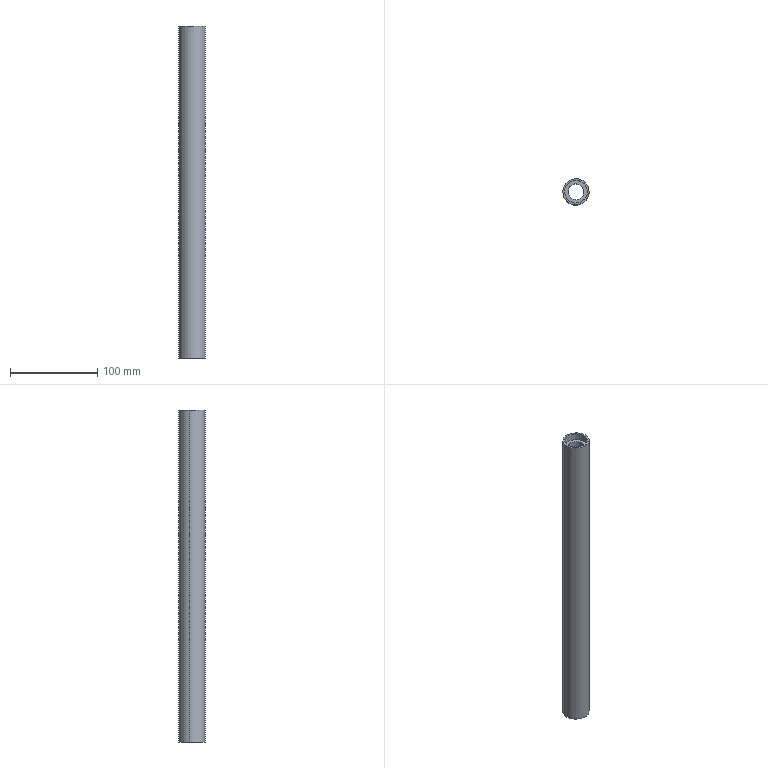Component | SolidWorks | Roller1-2-1_Roller1-1 | 1 solid | 12 faces | box 30 x 30 x 380 mm | volume 167485 mm3 | cylinder 8 | plane 4 | commonest cylinder face diameters 26 x4 18 x2 30 x2
build123d program:
from build123d import *


with BuildPart() as part:
    # Sketch1 → Revolve1 (revolve)
    with BuildSketch(Plane(origin=(0, 0, 0), x_dir=(-1, 0, 0), z_dir=(0, 0, -1)), mode=Mode.PRIVATE) as revolve1_sk:
        Polygon((-182, 13), (-182, 9), (182, 9), (182, 13), (190, 13), (190, 15), (-190, 15), (-190, 13), align=None)
    revolve(revolve1_sk.sketch.rotate(Axis((190, 0, 0), (-1, 0, 0)), 270), axis=Axis((190, 0, 0), (-1, 0, 0)))


solid = part.part

# Placed as in the assembly
solid = solid.moved(Location((-365, 591, 0), (0, 90, 0)))
STEP:
#1=CARTESIAN_POINT('',(-14.024,23.192,-7.165));
#2=VERTEX_POINT('',#1);
#3=CARTESIAN_POINT('',(-14.716,23.344,-7.165));
#4=VERTEX_POINT('',#3);
#5=CARTESIAN_POINT('',(-14.37,23.268,-7.165));
#6=DIRECTION('',(-0.,0.,1.));
#7=DIRECTION('',(-0.9768,0.2142,0.));
#8=AXIS2_PLACEMENT_3D('',#5,#6,#7);
#9=CIRCLE('',#8,0.3543);
#10=EDGE_CURVE('',#2,#4,#9,.T.);
#11=ORIENTED_EDGE('',*,*,#10,.F.);
#12=CARTESIAN_POINT('',(-14.024,23.192,7.165));
#13=VERTEX_POINT('',#12);
#14=CARTESIAN_POINT('',(-14.024,23.192,-7.48));
#15=DIRECTION('',(-0.,0.,1.));
#16=VECTOR('',#15,39.37);
#17=LINE('',#14,#16);
#18=EDGE_CURVE('',#2,#13,#17,.T.);
#19=ORIENTED_EDGE('',*,*,#18,.T.);
#20=CARTESIAN_POINT('',(-14.716,23.344,7.165));
#21=VERTEX_POINT('',#20);
#22=CARTESIAN_POINT('',(-14.37,23.268,7.165));
#23=DIRECTION('',(-0.,0.,1.));
#24=DIRECTION('',(-0.9768,0.2142,0.));
#25=AXIS2_PLACEMENT_3D('',#22,#23,#24);
#26=CIRCLE('',#25,0.3543);
#27=EDGE_CURVE('',#13,#21,#26,.T.);
#28=ORIENTED_EDGE('',*,*,#27,.T.);
#29=CARTESIAN_POINT('',(-14.716,23.344,-7.48));
#30=DIRECTION('',(-0.,0.,1.));
#31=VECTOR('',#30,39.37);
#32=LINE('',#29,#31);
#33=EDGE_CURVE('',#4,#21,#32,.T.);
#34=ORIENTED_EDGE('',*,*,#33,.F.);
#35=EDGE_LOOP('',(#11,#19,#28,#34));
#36=FACE_OUTER_BOUND('',#35,.T.);
#37=CARTESIAN_POINT('',(-14.37,23.268,-7.48));
#38=DIRECTION('',(-0.,0.,1.));
#39=DIRECTION('',(-0.9768,0.2142,0.));
#40=AXIS2_PLACEMENT_3D('',#37,#38,#39);
#41=CYLINDRICAL_SURFACE('',#40,0.3543);
#42=ADVANCED_FACE('',(#36),#41,.F.);
#43=CARTESIAN_POINT('',(-13.87,23.158,7.165));
#44=VERTEX_POINT('',#43);
#45=CARTESIAN_POINT('',(-14.87,23.377,7.165));
#46=VERTEX_POINT('',#45);
#47=CARTESIAN_POINT('',(-14.37,23.268,7.165));
#48=DIRECTION('',(-0.,0.,1.));
#49=DIRECTION('',(-0.9768,0.2142,0.));
#50=AXIS2_PLACEMENT_3D('',#47,#48,#49);
#51=CIRCLE('',#50,0.5118);
#52=EDGE_CURVE('',#44,#46,#51,.T.);
#53=ORIENTED_EDGE('',*,*,#52,.F.);
#54=CARTESIAN_POINT('',(-13.87,23.158,7.48));
#55=VERTEX_POINT('',#54);
#56=CARTESIAN_POINT('',(-13.87,23.158,-7.48));
#57=DIRECTION('',(-0.,0.,1.));
#58=VECTOR('',#57,39.37);
#59=LINE('',#56,#58);
#60=EDGE_CURVE('',#44,#55,#59,.T.);
#61=ORIENTED_EDGE('',*,*,#60,.T.);
#62=CARTESIAN_POINT('',(-14.87,23.377,7.48));
#63=VERTEX_POINT('',#62);
#64=CARTESIAN_POINT('',(-14.37,23.268,7.48));
#65=DIRECTION('',(-0.,0.,1.));
#66=DIRECTION('',(-0.9768,0.2142,0.));
#67=AXIS2_PLACEMENT_3D('',#64,#65,#66);
#68=CIRCLE('',#67,0.5118);
#69=EDGE_CURVE('',#55,#63,#68,.T.);
#70=ORIENTED_EDGE('',*,*,#69,.T.);
#71=CARTESIAN_POINT('',(-14.87,23.377,-7.48));
#72=DIRECTION('',(-0.,0.,1.));
#73=VECTOR('',#72,39.37);
#74=LINE('',#71,#73);
#75=EDGE_CURVE('',#46,#63,#74,.T.);
#76=ORIENTED_EDGE('',*,*,#75,.F.);
#77=EDGE_LOOP('',(#53,#61,#70,#76));
#78=FACE_OUTER_BOUND('',#77,.T.);
#79=CARTESIAN_POINT('',(-14.37,23.268,-7.48));
#80=DIRECTION('',(-0.,0.,1.));
#81=DIRECTION('',(-0.9768,0.2142,0.));
#82=AXIS2_PLACEMENT_3D('',#79,#80,#81);
#83=CYLINDRICAL_SURFACE('',#82,0.5118);
#84=ADVANCED_FACE('',(#78),#83,.F.);
#85=CARTESIAN_POINT('',(-14.947,23.394,-7.48));
#86=VERTEX_POINT('',#85);
#87=CARTESIAN_POINT('',(-13.793,23.141,-7.48));
#88=VERTEX_POINT('',#87);
#89=CARTESIAN_POINT('',(-14.37,23.268,-7.48));
#90=DIRECTION('',(-0.,0.,1.));
#91=DIRECTION('',(-0.9768,0.2142,0.));
#92=AXIS2_PLACEMENT_3D('',#89,#90,#91);
#93=CIRCLE('',#92,0.5906);
#94=EDGE_CURVE('',#86,#88,#93,.T.);
#95=ORIENTED_EDGE('',*,*,#94,.T.);
#96=CARTESIAN_POINT('',(-13.793,23.141,7.48));
#97=VERTEX_POINT('',#96);
#98=CARTESIAN_POINT('',(-13.793,23.141,-7.48));
#99=DIRECTION('',(-0.,0.,1.));
#100=VECTOR('',#99,39.37);
#101=LINE('',#98,#100);
#102=EDGE_CURVE('',#88,#97,#101,.T.);
#103=ORIENTED_EDGE('',*,*,#102,.T.);
#104=CARTESIAN_POINT('',(-14.947,23.394,7.48));
#105=VERTEX_POINT('',#104);
#106=CARTESIAN_POINT('',(-14.37,23.268,7.48));
#107=DIRECTION('',(-0.,0.,1.));
#108=DIRECTION('',(-0.9768,0.2142,0.));
#109=AXIS2_PLACEMENT_3D('',#106,#107,#108);
#110=CIRCLE('',#109,0.5906);
#111=EDGE_CURVE('',#105,#97,#110,.T.);
#112=ORIENTED_EDGE('',*,*,#111,.F.);
#113=CARTESIAN_POINT('',(-14.947,23.394,-7.48));
#114=DIRECTION('',(-0.,0.,1.));
#115=VECTOR('',#114,39.37);
#116=LINE('',#113,#115);
#117=EDGE_CURVE('',#86,#105,#116,.T.);
#118=ORIENTED_EDGE('',*,*,#117,.F.);
#119=EDGE_LOOP('',(#95,#103,#112,#118));
#120=FACE_OUTER_BOUND('',#119,.T.);
#121=CARTESIAN_POINT('',(-14.37,23.268,-7.48));
#122=DIRECTION('',(-0.,0.,1.));
#123=DIRECTION('',(-0.9768,0.2142,0.));
#124=AXIS2_PLACEMENT_3D('',#121,#122,#123);
#125=CYLINDRICAL_SURFACE('',#124,0.5906);
#126=ADVANCED_FACE('',(#120),#125,.T.);
#127=CARTESIAN_POINT('',(-13.87,23.158,-7.48));
#128=VERTEX_POINT('',#127);
#129=CARTESIAN_POINT('',(-14.87,23.377,-7.48));
#130=VERTEX_POINT('',#129);
#131=CARTESIAN_POINT('',(-14.37,23.268,-7.48));
#132=DIRECTION('',(-0.,0.,1.));
#133=DIRECTION('',(-0.9768,0.2142,0.));
#134=AXIS2_PLACEMENT_3D('',#131,#132,#133);
#135=CIRCLE('',#134,0.5118);
#136=EDGE_CURVE('',#128,#130,#135,.T.);
#137=ORIENTED_EDGE('',*,*,#136,.F.);
#138=CARTESIAN_POINT('',(-13.87,23.158,-7.165));
#139=VERTEX_POINT('',#138);
#140=CARTESIAN_POINT('',(-13.87,23.158,-7.48));
#141=DIRECTION('',(-0.,0.,1.));
#142=VECTOR('',#141,39.37);
#143=LINE('',#140,#142);
#144=EDGE_CURVE('',#128,#139,#143,.T.);
#145=ORIENTED_EDGE('',*,*,#144,.T.);
#146=CARTESIAN_POINT('',(-14.87,23.377,-7.165));
#147=VERTEX_POINT('',#146);
#148=CARTESIAN_POINT('',(-14.37,23.268,-7.165));
#149=DIRECTION('',(-0.,0.,1.));
#150=DIRECTION('',(-0.9768,0.2142,0.));
#151=AXIS2_PLACEMENT_3D('',#148,#149,#150);
#152=CIRCLE('',#151,0.5118);
#153=EDGE_CURVE('',#139,#147,#152,.T.);
#154=ORIENTED_EDGE('',*,*,#153,.T.);
#155=CARTESIAN_POINT('',(-14.87,23.377,-7.48));
#156=DIRECTION('',(-0.,0.,1.));
#157=VECTOR('',#156,39.37);
#158=LINE('',#155,#157);
#159=EDGE_CURVE('',#130,#147,#158,.T.);
#160=ORIENTED_EDGE('',*,*,#159,.F.);
#161=EDGE_LOOP('',(#137,#145,#154,#160));
#162=FACE_OUTER_BOUND('',#161,.T.);
#163=CARTESIAN_POINT('',(-14.37,23.268,-7.48));
#164=DIRECTION('',(-0.,0.,1.));
#165=DIRECTION('',(-0.9768,0.2142,0.));
#166=AXIS2_PLACEMENT_3D('',#163,#164,#165);
#167=CYLINDRICAL_SURFACE('',#166,0.5118);
#168=ADVANCED_FACE('',(#162),#167,.F.);
#169=ORIENTED_EDGE('',*,*,#144,.F.);
#170=CARTESIAN_POINT('',(-14.37,23.268,-7.48));
#171=DIRECTION('',(-0.,0.,1.));
#172=DIRECTION('',(-0.9768,0.2142,0.));
#173=AXIS2_PLACEMENT_3D('',#170,#171,#172);
#174=CIRCLE('',#173,0.5118);
#175=EDGE_CURVE('',#130,#128,#174,.T.);
#176=ORIENTED_EDGE('',*,*,#175,.F.);
#177=ORIENTED_EDGE('',*,*,#159,.T.);
#178=CARTESIAN_POINT('',(-14.37,23.268,-7.165));
#179=DIRECTION('',(-0.,0.,1.));
#180=DIRECTION('',(-0.9768,0.2142,0.));
#181=AXIS2_PLACEMENT_3D('',#178,#179,#180);
#182=CIRCLE('',#181,0.5118);
#183=EDGE_CURVE('',#147,#139,#182,.T.);
#184=ORIENTED_EDGE('',*,*,#183,.T.);
#185=EDGE_LOOP('',(#169,#176,#177,#184));
#186=FACE_OUTER_BOUND('',#185,.T.);
#187=CARTESIAN_POINT('',(-14.37,23.268,-7.48));
#188=DIRECTION('',(-0.,0.,1.));
#189=DIRECTION('',(-0.9768,0.2142,0.));
#190=AXIS2_PLACEMENT_3D('',#187,#188,#189);
#191=CYLINDRICAL_SURFACE('',#190,0.5118);
#192=ADVANCED_FACE('',(#186),#191,.F.);
#193=ORIENTED_EDGE('',*,*,#175,.T.);
#194=ORIENTED_EDGE('',*,*,#136,.T.);
#195=EDGE_LOOP('',(#193,#194));
#196=FACE_BOUND('',#195,.T.);
#197=ORIENTED_EDGE('',*,*,#94,.F.);
#198=CARTESIAN_POINT('',(-14.37,23.268,-7.48));
#199=DIRECTION('',(-0.,0.,1.));
#200=DIRECTION('',(-0.9768,0.2142,0.));
#201=AXIS2_PLACEMENT_3D('',#198,#199,#200);
#202=CIRCLE('',#201,0.5906);
#203=EDGE_CURVE('',#88,#86,#202,.T.);
#204=ORIENTED_EDGE('',*,*,#203,.F.);
#205=EDGE_LOOP('',(#197,#204));
#206=FACE_OUTER_BOUND('',#205,.T.);
#207=CARTESIAN_POINT('',(-14.497,22.691,-7.48));
#208=DIRECTION('',(0.,-0.,-1.));
#209=DIRECTION('',(0.9768,-0.2142,0.));
#210=AXIS2_PLACEMENT_3D('',#207,#208,#209);
#211=PLANE('',#210);
#212=ADVANCED_FACE('',(#196,#206),#211,.T.);
#213=ORIENTED_EDGE('',*,*,#102,.F.);
#214=ORIENTED_EDGE('',*,*,#203,.T.);
#215=ORIENTED_EDGE('',*,*,#117,.T.);
#216=CARTESIAN_POINT('',(-14.37,23.268,7.48));
#217=DIRECTION('',(-0.,0.,1.));
#218=DIRECTION('',(-0.9768,0.2142,0.));
#219=AXIS2_PLACEMENT_3D('',#216,#217,#218);
#220=CIRCLE('',#219,0.5906);
#221=EDGE_CURVE('',#97,#105,#220,.T.);
#222=ORIENTED_EDGE('',*,*,#221,.F.);
#223=EDGE_LOOP('',(#213,#214,#215,#222));
#224=FACE_OUTER_BOUND('',#223,.T.);
#225=CARTESIAN_POINT('',(-14.37,23.268,-7.48));
#226=DIRECTION('',(-0.,0.,1.));
#227=DIRECTION('',(-0.9768,0.2142,0.));
#228=AXIS2_PLACEMENT_3D('',#225,#226,#227);
#229=CYLINDRICAL_SURFACE('',#228,0.5906);
#230=ADVANCED_FACE('',(#224),#229,.T.);
#231=ORIENTED_EDGE('',*,*,#111,.T.);
#232=ORIENTED_EDGE('',*,*,#221,.T.);
#233=EDGE_LOOP('',(#231,#232));
#234=FACE_OUTER_BOUND('',#233,.T.);
#235=CARTESIAN_POINT('',(-14.37,23.268,7.48));
#236=DIRECTION('',(-0.,0.,1.));
#237=DIRECTION('',(-0.9768,0.2142,0.));
#238=AXIS2_PLACEMENT_3D('',#235,#236,#237);
#239=CIRCLE('',#238,0.5118);
#240=EDGE_CURVE('',#63,#55,#239,.T.);
#241=ORIENTED_EDGE('',*,*,#240,.F.);
#242=ORIENTED_EDGE('',*,*,#69,.F.);
#243=EDGE_LOOP('',(#241,#242));
#244=FACE_BOUND('',#243,.T.);
#245=CARTESIAN_POINT('',(-14.48,22.768,7.48));
#246=DIRECTION('',(-0.,0.,1.));
#247=DIRECTION('',(-0.9768,0.2142,-0.));
#248=AXIS2_PLACEMENT_3D('',#245,#246,#247);
#249=PLANE('',#248);
#250=ADVANCED_FACE('',(#234,#244),#249,.T.);
#251=ORIENTED_EDGE('',*,*,#60,.F.);
#252=CARTESIAN_POINT('',(-14.37,23.268,7.165));
#253=DIRECTION('',(-0.,0.,1.));
#254=DIRECTION('',(-0.9768,0.2142,0.));
#255=AXIS2_PLACEMENT_3D('',#252,#253,#254);
#256=CIRCLE('',#255,0.5118);
#257=EDGE_CURVE('',#46,#44,#256,.T.);
#258=ORIENTED_EDGE('',*,*,#257,.F.);
#259=ORIENTED_EDGE('',*,*,#75,.T.);
#260=ORIENTED_EDGE('',*,*,#240,.T.);
#261=EDGE_LOOP('',(#251,#258,#259,#260));
#262=FACE_OUTER_BOUND('',#261,.T.);
#263=CARTESIAN_POINT('',(-14.37,23.268,-7.48));
#264=DIRECTION('',(-0.,0.,1.));
#265=DIRECTION('',(-0.9768,0.2142,0.));
#266=AXIS2_PLACEMENT_3D('',#263,#264,#265);
#267=CYLINDRICAL_SURFACE('',#266,0.5118);
#268=ADVANCED_FACE('',(#262),#267,.F.);
#269=ORIENTED_EDGE('',*,*,#257,.T.);
#270=ORIENTED_EDGE('',*,*,#52,.T.);
#271=EDGE_LOOP('',(#269,#270));
#272=FACE_OUTER_BOUND('',#271,.T.);
#273=CARTESIAN_POINT('',(-14.37,23.268,7.165));
#274=DIRECTION('',(-0.,0.,1.));
#275=DIRECTION('',(-0.9768,0.2142,0.));
#276=AXIS2_PLACEMENT_3D('',#273,#274,#275);
#277=CIRCLE('',#276,0.3543);
#278=EDGE_CURVE('',#21,#13,#277,.T.);
#279=ORIENTED_EDGE('',*,*,#278,.F.);
#280=ORIENTED_EDGE('',*,*,#27,.F.);
#281=EDGE_LOOP('',(#279,#280));
#282=FACE_BOUND('',#281,.T.);
#283=CARTESIAN_POINT('',(-14.446,22.922,7.165));
#284=DIRECTION('',(-0.,0.,1.));
#285=DIRECTION('',(-0.9768,0.2142,-0.));
#286=AXIS2_PLACEMENT_3D('',#283,#284,#285);
#287=PLANE('',#286);
#288=ADVANCED_FACE('',(#272,#282),#287,.T.);
#289=ORIENTED_EDGE('',*,*,#18,.F.);
#290=CARTESIAN_POINT('',(-14.37,23.268,-7.165));
#291=DIRECTION('',(-0.,0.,1.));
#292=DIRECTION('',(-0.9768,0.2142,0.));
#293=AXIS2_PLACEMENT_3D('',#290,#291,#292);
#294=CIRCLE('',#293,0.3543);
#295=EDGE_CURVE('',#4,#2,#294,.T.);
#296=ORIENTED_EDGE('',*,*,#295,.F.);
#297=ORIENTED_EDGE('',*,*,#33,.T.);
#298=ORIENTED_EDGE('',*,*,#278,.T.);
#299=EDGE_LOOP('',(#289,#296,#297,#298));
#300=FACE_OUTER_BOUND('',#299,.T.);
#301=CARTESIAN_POINT('',(-14.37,23.268,-7.48));
#302=DIRECTION('',(-0.,0.,1.));
#303=DIRECTION('',(-0.9768,0.2142,0.));
#304=AXIS2_PLACEMENT_3D('',#301,#302,#303);
#305=CYLINDRICAL_SURFACE('',#304,0.3543);
#306=ADVANCED_FACE('',(#300),#305,.F.);
#307=ORIENTED_EDGE('',*,*,#295,.T.);
#308=ORIENTED_EDGE('',*,*,#10,.T.);
#309=EDGE_LOOP('',(#307,#308));
#310=FACE_BOUND('',#309,.T.);
#311=ORIENTED_EDGE('',*,*,#183,.F.);
#312=ORIENTED_EDGE('',*,*,#153,.F.);
#313=EDGE_LOOP('',(#311,#312));
#314=FACE_OUTER_BOUND('',#313,.T.);
#315=CARTESIAN_POINT('',(-14.48,22.768,-7.165));
#316=DIRECTION('',(0.,-0.,-1.));
#317=DIRECTION('',(0.9768,-0.2142,0.));
#318=AXIS2_PLACEMENT_3D('',#315,#316,#317);
#319=PLANE('',#318);
#320=ADVANCED_FACE('',(#310,#314),#319,.T.);
#321=CLOSED_SHELL('',(#42,#84,#126,#168,#192,#212,#230,#250,#268,#288,#306,#320));
#322=MANIFOLD_SOLID_BREP('',#321);
#323=CARTESIAN_POINT('',(0.,0.,0.));
#324=DIRECTION('',(0.,0.,1.));
#325=DIRECTION('',(1.,0.,0.));
#326=AXIS2_PLACEMENT_3D('',#323,#324,#325);
#327=(LENGTH_UNIT()NAMED_UNIT(*)SI_UNIT($,.METRE.));
#328=LENGTH_MEASURE_WITH_UNIT(LENGTH_MEASURE(0.0254),#327);
#329=DIMENSIONAL_EXPONENTS(1.,0.,0.,0.,0.,0.,0.);
#330=(CONVERSION_BASED_UNIT('',#328)LENGTH_UNIT()NAMED_UNIT(#329));
#331=UNCERTAINTY_MEASURE_WITH_UNIT(LENGTH_MEASURE(0.00001),#330,'','');
#332=(NAMED_UNIT(*)PLANE_ANGLE_UNIT()SI_UNIT($,.RADIAN.));
#333=(NAMED_UNIT(*)SI_UNIT($,.STERADIAN.)SOLID_ANGLE_UNIT());
#334=(GEOMETRIC_REPRESENTATION_CONTEXT(3)GLOBAL_UNCERTAINTY_ASSIGNED_CONTEXT((#331))GLOBAL_UNIT_ASSIGNED_CONTEXT((#330,#332,#333))REPRESENTATION_CONTEXT('',''));
#335=ADVANCED_BREP_SHAPE_REPRESENTATION('',(#322,#326),#334);
#336=COLOUR_RGB('',0.7922,0.8196,0.9333);
#337=FILL_AREA_STYLE_COLOUR('',#336);
#338=FILL_AREA_STYLE('',(#337));
#339=SURFACE_STYLE_FILL_AREA(#338);
#340=SURFACE_SIDE_STYLE('',(#339));
#341=SURFACE_STYLE_USAGE(.BOTH.,#340);
#342=PRESENTATION_STYLE_ASSIGNMENT((#341));
#343=STYLED_ITEM('',(#342),#322);
#344=PRESENTATION_LAYER_ASSIGNMENT('','',(#343));
#345=(LENGTH_UNIT()NAMED_UNIT(*)SI_UNIT($,.METRE.));
#346=LENGTH_MEASURE_WITH_UNIT(LENGTH_MEASURE(0.0254),#345);
#347=DIMENSIONAL_EXPONENTS(1.,0.,0.,0.,0.,0.,0.);
#348=(CONVERSION_BASED_UNIT('',#346)LENGTH_UNIT()NAMED_UNIT(#347));
#349=UNCERTAINTY_MEASURE_WITH_UNIT(LENGTH_MEASURE(0.00001),#348,'','');
#350=(NAMED_UNIT(*)PLANE_ANGLE_UNIT()SI_UNIT($,.RADIAN.));
#351=(NAMED_UNIT(*)SI_UNIT($,.STERADIAN.)SOLID_ANGLE_UNIT());
#352=(GEOMETRIC_REPRESENTATION_CONTEXT(3)GLOBAL_UNCERTAINTY_ASSIGNED_CONTEXT((#349))GLOBAL_UNIT_ASSIGNED_CONTEXT((#348,#350,#351))REPRESENTATION_CONTEXT('',''));
#353=MECHANICAL_DESIGN_GEOMETRIC_PRESENTATION_REPRESENTATION('',(#343),#352);